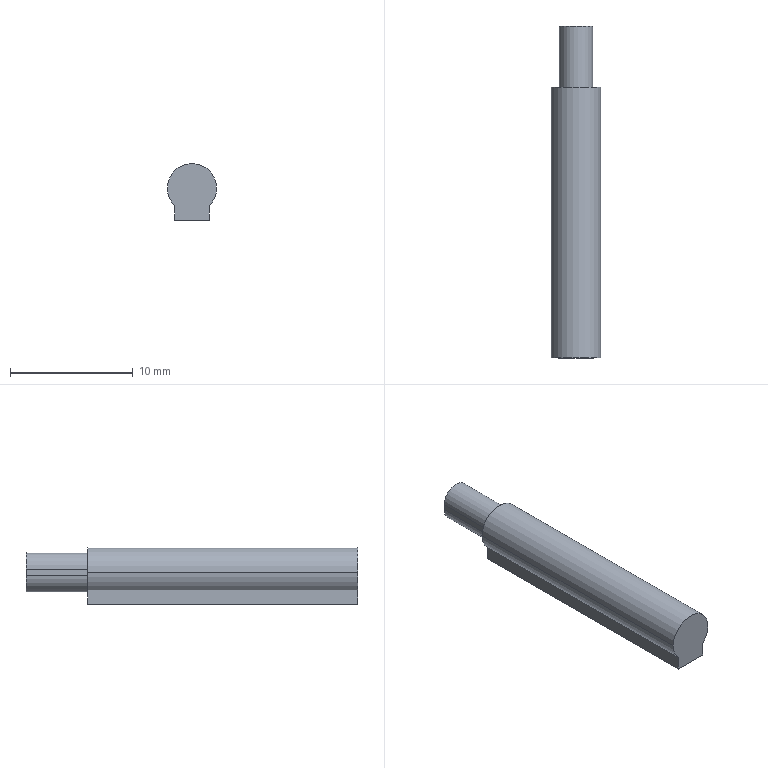Component | SolidWorks | RSDQA32-20DD-M9BL(0_0)-1_RSDQ_D-M9BL_SW(32)_2-1 | 1 solid | 16 faces | box 4 x 27 x 4.6 mm | volume 359 mm3 | plane 9 | cylinder 7 | commonest cylinder face diameters 4 x3 2.5 x2 2.7 x2
STEP:
#1=COLOUR_RGB('',0.7922,0.8196,0.9333);
#2=FILL_AREA_STYLE_COLOUR('',#1);
#3=FILL_AREA_STYLE('',(#2));
#4=SURFACE_STYLE_FILL_AREA(#3);
#5=SURFACE_SIDE_STYLE('',(#4));
#6=SURFACE_STYLE_USAGE(.BOTH.,#5);
#7=PRESENTATION_STYLE_ASSIGNMENT((#6));
#8=CARTESIAN_POINT('',(0.2128,-2.152,-1.666));
#9=VERTEX_POINT('',#8);
#10=CARTESIAN_POINT('',(0.1892,-2.152,-1.61));
#11=VERTEX_POINT('',#10);
#12=CARTESIAN_POINT('',(0.2679,-2.152,-1.61));
#13=DIRECTION('',(-0.,1.,0.));
#14=DIRECTION('',(1.,0.,0.));
#15=AXIS2_PLACEMENT_3D('',#12,#13,#14);
#16=CIRCLE('',#15,0.07874);
#17=EDGE_CURVE('',#9,#11,#16,.T.);
#18=ORIENTED_EDGE('',*,*,#17,.T.);
#19=CARTESIAN_POINT('',(0.1892,-1.286,-1.61));
#20=VERTEX_POINT('',#19);
#21=CARTESIAN_POINT('',(0.1892,-2.152,-1.61));
#22=DIRECTION('',(-0.,1.,0.));
#23=VECTOR('',#22,39.37);
#24=LINE('',#21,#23);
#25=EDGE_CURVE('',#11,#20,#24,.T.);
#26=ORIENTED_EDGE('',*,*,#25,.T.);
#27=CARTESIAN_POINT('',(0.2128,-1.286,-1.666));
#28=VERTEX_POINT('',#27);
#29=CARTESIAN_POINT('',(0.2679,-1.286,-1.61));
#30=DIRECTION('',(0.,-1.,-0.));
#31=DIRECTION('',(1.,0.,-0.));
#32=AXIS2_PLACEMENT_3D('',#29,#30,#31);
#33=CIRCLE('',#32,0.07874);
#34=EDGE_CURVE('',#20,#28,#33,.T.);
#35=ORIENTED_EDGE('',*,*,#34,.T.);
#36=CARTESIAN_POINT('',(0.2128,-2.152,-1.666));
#37=DIRECTION('',(0.,-1.,-0.));
#38=VECTOR('',#37,39.37);
#39=LINE('',#36,#38);
#40=EDGE_CURVE('',#28,#9,#39,.T.);
#41=ORIENTED_EDGE('',*,*,#40,.T.);
#42=EDGE_LOOP('',(#18,#26,#35,#41));
#43=FACE_OUTER_BOUND('',#42,.T.);
#44=CARTESIAN_POINT('',(0.2679,-2.152,-1.61));
#45=DIRECTION('',(-0.,1.,0.));
#46=DIRECTION('',(1.,0.,0.));
#47=AXIS2_PLACEMENT_3D('',#44,#45,#46);
#48=CYLINDRICAL_SURFACE('',#47,0.07874);
#49=ADVANCED_FACE('',(#43),#48,.T.);
#50=ORIENTED_EDGE('',*,*,#25,.F.);
#51=CARTESIAN_POINT('',(0.3466,-2.152,-1.61));
#52=VERTEX_POINT('',#51);
#53=CARTESIAN_POINT('',(0.2679,-2.152,-1.61));
#54=DIRECTION('',(-0.,1.,0.));
#55=DIRECTION('',(1.,0.,0.));
#56=AXIS2_PLACEMENT_3D('',#53,#54,#55);
#57=CIRCLE('',#56,0.07874);
#58=EDGE_CURVE('',#11,#52,#57,.T.);
#59=ORIENTED_EDGE('',*,*,#58,.T.);
#60=CARTESIAN_POINT('',(0.3466,-1.286,-1.61));
#61=VERTEX_POINT('',#60);
#62=CARTESIAN_POINT('',(0.3466,-2.152,-1.61));
#63=DIRECTION('',(-0.,1.,0.));
#64=VECTOR('',#63,39.37);
#65=LINE('',#62,#64);
#66=EDGE_CURVE('',#52,#61,#65,.T.);
#67=ORIENTED_EDGE('',*,*,#66,.T.);
#68=CARTESIAN_POINT('',(0.2679,-1.286,-1.61));
#69=DIRECTION('',(0.,-1.,-0.));
#70=DIRECTION('',(1.,0.,0.));
#71=AXIS2_PLACEMENT_3D('',#68,#69,#70);
#72=CIRCLE('',#71,0.07874);
#73=EDGE_CURVE('',#61,#20,#72,.T.);
#74=ORIENTED_EDGE('',*,*,#73,.T.);
#75=EDGE_LOOP('',(#50,#59,#67,#74));
#76=FACE_OUTER_BOUND('',#75,.T.);
#77=CARTESIAN_POINT('',(0.2679,-2.152,-1.61));
#78=DIRECTION('',(-0.,1.,0.));
#79=DIRECTION('',(1.,0.,0.));
#80=AXIS2_PLACEMENT_3D('',#77,#78,#79);
#81=CYLINDRICAL_SURFACE('',#80,0.07874);
#82=ADVANCED_FACE('',(#76),#81,.T.);
#83=CARTESIAN_POINT('',(0.3171,-2.073,-1.713));
#84=VERTEX_POINT('',#83);
#85=CARTESIAN_POINT('',(0.2187,-2.073,-1.713));
#86=VERTEX_POINT('',#85);
#87=CARTESIAN_POINT('',(0.2679,-2.073,-1.713));
#88=DIRECTION('',(0.,-0.,1.));
#89=DIRECTION('',(-1.,0.,0.));
#90=AXIS2_PLACEMENT_3D('',#87,#88,#89);
#91=CIRCLE('',#90,0.04921);
#92=EDGE_CURVE('',#84,#86,#91,.T.);
#93=ORIENTED_EDGE('',*,*,#92,.F.);
#94=CARTESIAN_POINT('',(0.3171,-2.073,-1.705));
#95=VERTEX_POINT('',#94);
#96=CARTESIAN_POINT('',(0.3171,-2.073,-1.713));
#97=DIRECTION('',(0.,-0.,1.));
#98=VECTOR('',#97,39.37);
#99=LINE('',#96,#98);
#100=EDGE_CURVE('',#84,#95,#99,.T.);
#101=ORIENTED_EDGE('',*,*,#100,.T.);
#102=CARTESIAN_POINT('',(0.2187,-2.073,-1.705));
#103=VERTEX_POINT('',#102);
#104=CARTESIAN_POINT('',(0.2679,-2.073,-1.705));
#105=DIRECTION('',(-0.,0.,-1.));
#106=DIRECTION('',(-1.,0.,0.));
#107=AXIS2_PLACEMENT_3D('',#104,#105,#106);
#108=CIRCLE('',#107,0.04921);
#109=EDGE_CURVE('',#103,#95,#108,.T.);
#110=ORIENTED_EDGE('',*,*,#109,.F.);
#111=CARTESIAN_POINT('',(0.2187,-2.073,-1.713));
#112=DIRECTION('',(0.,-0.,1.));
#113=VECTOR('',#112,39.37);
#114=LINE('',#111,#113);
#115=EDGE_CURVE('',#86,#103,#114,.T.);
#116=ORIENTED_EDGE('',*,*,#115,.F.);
#117=EDGE_LOOP('',(#93,#101,#110,#116));
#118=FACE_OUTER_BOUND('',#117,.T.);
#119=CARTESIAN_POINT('',(0.2679,-2.073,-1.713));
#120=DIRECTION('',(0.,-0.,1.));
#121=DIRECTION('',(-1.,0.,0.));
#122=AXIS2_PLACEMENT_3D('',#119,#120,#121);
#123=CYLINDRICAL_SURFACE('',#122,0.04921);
#124=ADVANCED_FACE('',(#118),#123,.F.);
#125=ORIENTED_EDGE('',*,*,#66,.F.);
#126=CARTESIAN_POINT('',(0.323,-2.152,-1.666));
#127=VERTEX_POINT('',#126);
#128=CARTESIAN_POINT('',(0.2679,-2.152,-1.61));
#129=DIRECTION('',(-0.,1.,0.));
#130=DIRECTION('',(1.,0.,0.));
#131=AXIS2_PLACEMENT_3D('',#128,#129,#130);
#132=CIRCLE('',#131,0.07874);
#133=EDGE_CURVE('',#52,#127,#132,.T.);
#134=ORIENTED_EDGE('',*,*,#133,.T.);
#135=CARTESIAN_POINT('',(0.323,-1.286,-1.666));
#136=VERTEX_POINT('',#135);
#137=CARTESIAN_POINT('',(0.323,-2.152,-1.666));
#138=DIRECTION('',(-0.,1.,0.));
#139=VECTOR('',#138,39.37);
#140=LINE('',#137,#139);
#141=EDGE_CURVE('',#127,#136,#140,.T.);
#142=ORIENTED_EDGE('',*,*,#141,.T.);
#143=CARTESIAN_POINT('',(0.2679,-1.286,-1.61));
#144=DIRECTION('',(0.,-1.,-0.));
#145=DIRECTION('',(1.,0.,-0.));
#146=AXIS2_PLACEMENT_3D('',#143,#144,#145);
#147=CIRCLE('',#146,0.07874);
#148=EDGE_CURVE('',#136,#61,#147,.T.);
#149=ORIENTED_EDGE('',*,*,#148,.T.);
#150=EDGE_LOOP('',(#125,#134,#142,#149));
#151=FACE_OUTER_BOUND('',#150,.T.);
#152=CARTESIAN_POINT('',(0.2679,-2.152,-1.61));
#153=DIRECTION('',(-0.,1.,0.));
#154=DIRECTION('',(1.,0.,0.));
#155=AXIS2_PLACEMENT_3D('',#152,#153,#154);
#156=CYLINDRICAL_SURFACE('',#155,0.07874);
#157=ADVANCED_FACE('',(#151),#156,.T.);
#158=CARTESIAN_POINT('',(0.323,-2.152,-1.713));
#159=VERTEX_POINT('',#158);
#160=CARTESIAN_POINT('',(0.323,-2.152,-1.713));
#161=DIRECTION('',(-0.,0.,-1.));
#162=VECTOR('',#161,39.37);
#163=LINE('',#160,#162);
#164=EDGE_CURVE('',#127,#159,#163,.T.);
#165=ORIENTED_EDGE('',*,*,#164,.T.);
#166=CARTESIAN_POINT('',(0.323,-1.286,-1.713));
#167=VERTEX_POINT('',#166);
#168=CARTESIAN_POINT('',(0.323,-2.152,-1.713));
#169=DIRECTION('',(-0.,1.,0.));
#170=VECTOR('',#169,39.37);
#171=LINE('',#168,#170);
#172=EDGE_CURVE('',#159,#167,#171,.T.);
#173=ORIENTED_EDGE('',*,*,#172,.T.);
#174=CARTESIAN_POINT('',(0.323,-1.286,-1.713));
#175=DIRECTION('',(0.,-0.,1.));
#176=VECTOR('',#175,39.37);
#177=LINE('',#174,#176);
#178=EDGE_CURVE('',#167,#136,#177,.T.);
#179=ORIENTED_EDGE('',*,*,#178,.T.);
#180=ORIENTED_EDGE('',*,*,#141,.F.);
#181=EDGE_LOOP('',(#165,#173,#179,#180));
#182=FACE_OUTER_BOUND('',#181,.T.);
#183=CARTESIAN_POINT('',(0.323,-2.152,-1.713));
#184=DIRECTION('',(1.,0.,-0.));
#185=DIRECTION('',(0.,-1.,-0.));
#186=AXIS2_PLACEMENT_3D('',#183,#184,#185);
#187=PLANE('',#186);
#188=ADVANCED_FACE('',(#182),#187,.T.);
#189=CARTESIAN_POINT('',(0.2128,-2.152,-1.713));
#190=VERTEX_POINT('',#189);
#191=CARTESIAN_POINT('',(0.2128,-2.152,-1.61));
#192=DIRECTION('',(0.,-0.,1.));
#193=VECTOR('',#192,39.37);
#194=LINE('',#191,#193);
#195=EDGE_CURVE('',#190,#9,#194,.T.);
#196=ORIENTED_EDGE('',*,*,#195,.F.);
#197=CARTESIAN_POINT('',(0.2679,-2.152,-1.713));
#198=DIRECTION('',(-1.,-0.,0.));
#199=VECTOR('',#198,39.37);
#200=LINE('',#197,#199);
#201=EDGE_CURVE('',#159,#190,#200,.T.);
#202=ORIENTED_EDGE('',*,*,#201,.F.);
#203=ORIENTED_EDGE('',*,*,#164,.F.);
#204=ORIENTED_EDGE('',*,*,#133,.F.);
#205=ORIENTED_EDGE('',*,*,#58,.F.);
#206=ORIENTED_EDGE('',*,*,#17,.F.);
#207=EDGE_LOOP('',(#196,#202,#203,#204,#205,#206));
#208=FACE_OUTER_BOUND('',#207,.T.);
#209=CARTESIAN_POINT('',(0.2679,-2.152,-1.61));
#210=DIRECTION('',(-0.,1.,0.));
#211=DIRECTION('',(1.,0.,-0.));
#212=AXIS2_PLACEMENT_3D('',#209,#210,#211);
#213=PLANE('',#212);
#214=ADVANCED_FACE('',(#208),#213,.F.);
#215=ORIENTED_EDGE('',*,*,#195,.T.);
#216=ORIENTED_EDGE('',*,*,#40,.F.);
#217=CARTESIAN_POINT('',(0.2128,-1.286,-1.713));
#218=VERTEX_POINT('',#217);
#219=CARTESIAN_POINT('',(0.2128,-1.286,-1.666));
#220=DIRECTION('',(-0.,0.,-1.));
#221=VECTOR('',#220,39.37);
#222=LINE('',#219,#221);
#223=EDGE_CURVE('',#28,#218,#222,.T.);
#224=ORIENTED_EDGE('',*,*,#223,.T.);
#225=CARTESIAN_POINT('',(0.2128,-2.152,-1.713));
#226=DIRECTION('',(0.,-1.,-0.));
#227=VECTOR('',#226,39.37);
#228=LINE('',#225,#227);
#229=EDGE_CURVE('',#218,#190,#228,.T.);
#230=ORIENTED_EDGE('',*,*,#229,.T.);
#231=EDGE_LOOP('',(#215,#216,#224,#230));
#232=FACE_OUTER_BOUND('',#231,.T.);
#233=CARTESIAN_POINT('',(0.2128,-2.152,-1.666));
#234=DIRECTION('',(-1.,-0.,0.));
#235=DIRECTION('',(-0.,1.,0.));
#236=AXIS2_PLACEMENT_3D('',#233,#234,#235);
#237=PLANE('',#236);
#238=ADVANCED_FACE('',(#232),#237,.T.);
#239=ORIENTED_EDGE('',*,*,#178,.F.);
#240=CARTESIAN_POINT('',(0.2679,-1.286,-1.713));
#241=DIRECTION('',(-1.,-0.,0.));
#242=VECTOR('',#241,39.37);
#243=LINE('',#240,#242);
#244=EDGE_CURVE('',#167,#218,#243,.T.);
#245=ORIENTED_EDGE('',*,*,#244,.T.);
#246=ORIENTED_EDGE('',*,*,#223,.F.);
#247=ORIENTED_EDGE('',*,*,#34,.F.);
#248=ORIENTED_EDGE('',*,*,#73,.F.);
#249=ORIENTED_EDGE('',*,*,#148,.F.);
#250=EDGE_LOOP('',(#239,#245,#246,#247,#248,#249));
#251=FACE_OUTER_BOUND('',#250,.T.);
#252=CARTESIAN_POINT('',(0.3211,-1.286,-1.6));
#253=VERTEX_POINT('',#252);
#254=CARTESIAN_POINT('',(0.3211,-1.286,-1.62));
#255=VERTEX_POINT('',#254);
#256=CARTESIAN_POINT('',(0.3211,-1.286,-1.62));
#257=DIRECTION('',(-0.,0.,-1.));
#258=VECTOR('',#257,39.37);
#259=LINE('',#256,#258);
#260=EDGE_CURVE('',#253,#255,#259,.T.);
#261=ORIENTED_EDGE('',*,*,#260,.F.);
#262=CARTESIAN_POINT('',(0.2148,-1.286,-1.6));
#263=VERTEX_POINT('',#262);
#264=CARTESIAN_POINT('',(0.2679,-1.286,-1.6));
#265=DIRECTION('',(0.,-1.,-0.));
#266=DIRECTION('',(1.,0.,0.));
#267=AXIS2_PLACEMENT_3D('',#264,#265,#266);
#268=CIRCLE('',#267,0.05315);
#269=EDGE_CURVE('',#253,#263,#268,.T.);
#270=ORIENTED_EDGE('',*,*,#269,.T.);
#271=CARTESIAN_POINT('',(0.2148,-1.286,-1.62));
#272=VERTEX_POINT('',#271);
#273=CARTESIAN_POINT('',(0.2148,-1.286,-1.6));
#274=DIRECTION('',(0.,-0.,1.));
#275=VECTOR('',#274,39.37);
#276=LINE('',#273,#275);
#277=EDGE_CURVE('',#272,#263,#276,.T.);
#278=ORIENTED_EDGE('',*,*,#277,.F.);
#279=CARTESIAN_POINT('',(0.2679,-1.286,-1.62));
#280=DIRECTION('',(0.,-1.,-0.));
#281=DIRECTION('',(1.,0.,0.));
#282=AXIS2_PLACEMENT_3D('',#279,#280,#281);
#283=CIRCLE('',#282,0.05315);
#284=EDGE_CURVE('',#272,#255,#283,.T.);
#285=ORIENTED_EDGE('',*,*,#284,.T.);
#286=EDGE_LOOP('',(#261,#270,#278,#285));
#287=FACE_BOUND('',#286,.T.);
#288=CARTESIAN_POINT('',(0.2679,-1.286,-1.61));
#289=DIRECTION('',(-0.,1.,0.));
#290=DIRECTION('',(1.,0.,-0.));
#291=AXIS2_PLACEMENT_3D('',#288,#289,#290);
#292=PLANE('',#291);
#293=ADVANCED_FACE('',(#251,#287),#292,.T.);
#294=ORIENTED_EDGE('',*,*,#201,.T.);
#295=ORIENTED_EDGE('',*,*,#229,.F.);
#296=ORIENTED_EDGE('',*,*,#244,.F.);
#297=ORIENTED_EDGE('',*,*,#172,.F.);
#298=EDGE_LOOP('',(#294,#295,#296,#297));
#299=FACE_OUTER_BOUND('',#298,.T.);
#300=CARTESIAN_POINT('',(0.2679,-2.073,-1.713));
#301=DIRECTION('',(0.,-0.,1.));
#302=DIRECTION('',(-1.,0.,0.));
#303=AXIS2_PLACEMENT_3D('',#300,#301,#302);
#304=CIRCLE('',#303,0.04921);
#305=EDGE_CURVE('',#86,#84,#304,.T.);
#306=ORIENTED_EDGE('',*,*,#305,.T.);
#307=ORIENTED_EDGE('',*,*,#92,.T.);
#308=EDGE_LOOP('',(#306,#307));
#309=FACE_BOUND('',#308,.T.);
#310=CARTESIAN_POINT('',(0.2128,-2.152,-1.713));
#311=DIRECTION('',(-0.,0.,-1.));
#312=DIRECTION('',(1.,0.,-0.));
#313=AXIS2_PLACEMENT_3D('',#310,#311,#312);
#314=PLANE('',#313);
#315=ADVANCED_FACE('',(#299,#309),#314,.T.);
#316=CARTESIAN_POINT('',(0.3211,-1.089,-1.6));
#317=VERTEX_POINT('',#316);
#318=CARTESIAN_POINT('',(0.2148,-1.089,-1.6));
#319=VERTEX_POINT('',#318);
#320=CARTESIAN_POINT('',(0.2679,-1.089,-1.6));
#321=DIRECTION('',(0.,-1.,-0.));
#322=DIRECTION('',(1.,0.,0.));
#323=AXIS2_PLACEMENT_3D('',#320,#321,#322);
#324=CIRCLE('',#323,0.05315);
#325=EDGE_CURVE('',#317,#319,#324,.T.);
#326=ORIENTED_EDGE('',*,*,#325,.T.);
#327=CARTESIAN_POINT('',(0.2148,-2.152,-1.6));
#328=DIRECTION('',(0.,-1.,-0.));
#329=VECTOR('',#328,39.37);
#330=LINE('',#327,#329);
#331=EDGE_CURVE('',#319,#263,#330,.T.);
#332=ORIENTED_EDGE('',*,*,#331,.T.);
#333=ORIENTED_EDGE('',*,*,#269,.F.);
#334=CARTESIAN_POINT('',(0.3211,-2.152,-1.6));
#335=DIRECTION('',(-0.,1.,0.));
#336=VECTOR('',#335,39.37);
#337=LINE('',#334,#336);
#338=EDGE_CURVE('',#253,#317,#337,.T.);
#339=ORIENTED_EDGE('',*,*,#338,.T.);
#340=EDGE_LOOP('',(#326,#332,#333,#339));
#341=FACE_OUTER_BOUND('',#340,.T.);
#342=CARTESIAN_POINT('',(0.2679,-2.152,-1.6));
#343=DIRECTION('',(-0.,1.,0.));
#344=DIRECTION('',(1.,0.,0.));
#345=AXIS2_PLACEMENT_3D('',#342,#343,#344);
#346=CYLINDRICAL_SURFACE('',#345,0.05315);
#347=ADVANCED_FACE('',(#341),#346,.T.);
#348=CARTESIAN_POINT('',(0.2148,-1.089,-1.62));
#349=VERTEX_POINT('',#348);
#350=CARTESIAN_POINT('',(0.3211,-1.089,-1.62));
#351=VERTEX_POINT('',#350);
#352=CARTESIAN_POINT('',(0.2679,-1.089,-1.62));
#353=DIRECTION('',(0.,-1.,-0.));
#354=DIRECTION('',(1.,0.,0.));
#355=AXIS2_PLACEMENT_3D('',#352,#353,#354);
#356=CIRCLE('',#355,0.05315);
#357=EDGE_CURVE('',#349,#351,#356,.T.);
#358=ORIENTED_EDGE('',*,*,#357,.T.);
#359=CARTESIAN_POINT('',(0.3211,-2.152,-1.62));
#360=DIRECTION('',(0.,-1.,-0.));
#361=VECTOR('',#360,39.37);
#362=LINE('',#359,#361);
#363=EDGE_CURVE('',#351,#255,#362,.T.);
#364=ORIENTED_EDGE('',*,*,#363,.T.);
#365=ORIENTED_EDGE('',*,*,#284,.F.);
#366=CARTESIAN_POINT('',(0.2148,-2.152,-1.62));
#367=DIRECTION('',(-0.,1.,0.));
#368=VECTOR('',#367,39.37);
#369=LINE('',#366,#368);
#370=EDGE_CURVE('',#272,#349,#369,.T.);
#371=ORIENTED_EDGE('',*,*,#370,.T.);
#372=EDGE_LOOP('',(#358,#364,#365,#371));
#373=FACE_OUTER_BOUND('',#372,.T.);
#374=CARTESIAN_POINT('',(0.2679,-2.152,-1.62));
#375=DIRECTION('',(-0.,1.,0.));
#376=DIRECTION('',(1.,0.,0.));
#377=AXIS2_PLACEMENT_3D('',#374,#375,#376);
#378=CYLINDRICAL_SURFACE('',#377,0.05315);
#379=ADVANCED_FACE('',(#373),#378,.T.);
#380=ORIENTED_EDGE('',*,*,#100,.F.);
#381=ORIENTED_EDGE('',*,*,#305,.F.);
#382=ORIENTED_EDGE('',*,*,#115,.T.);
#383=CARTESIAN_POINT('',(0.2679,-2.073,-1.705));
#384=DIRECTION('',(-0.,0.,-1.));
#385=DIRECTION('',(-1.,0.,0.));
#386=AXIS2_PLACEMENT_3D('',#383,#384,#385);
#387=CIRCLE('',#386,0.04921);
#388=EDGE_CURVE('',#95,#103,#387,.T.);
#389=ORIENTED_EDGE('',*,*,#388,.F.);
#390=EDGE_LOOP('',(#380,#381,#382,#389));
#391=FACE_OUTER_BOUND('',#390,.T.);
#392=CARTESIAN_POINT('',(0.2679,-2.073,-1.713));
#393=DIRECTION('',(0.,-0.,1.));
#394=DIRECTION('',(-1.,0.,0.));
#395=AXIS2_PLACEMENT_3D('',#392,#393,#394);
#396=CYLINDRICAL_SURFACE('',#395,0.04921);
#397=ADVANCED_FACE('',(#391),#396,.F.);
#398=CARTESIAN_POINT('',(0.2148,-1.089,-1.6));
#399=DIRECTION('',(-0.,0.,-1.));
#400=VECTOR('',#399,39.37);
#401=LINE('',#398,#400);
#402=EDGE_CURVE('',#319,#349,#401,.T.);
#403=ORIENTED_EDGE('',*,*,#402,.T.);
#404=ORIENTED_EDGE('',*,*,#370,.F.);
#405=ORIENTED_EDGE('',*,*,#277,.T.);
#406=ORIENTED_EDGE('',*,*,#331,.F.);
#407=EDGE_LOOP('',(#403,#404,#405,#406));
#408=FACE_OUTER_BOUND('',#407,.T.);
#409=CARTESIAN_POINT('',(0.2148,-2.152,-1.6));
#410=DIRECTION('',(-1.,-0.,0.));
#411=DIRECTION('',(-0.,1.,0.));
#412=AXIS2_PLACEMENT_3D('',#409,#410,#411);
#413=PLANE('',#412);
#414=ADVANCED_FACE('',(#408),#413,.T.);
#415=CARTESIAN_POINT('',(0.3211,-1.089,-1.61));
#416=DIRECTION('',(-0.,0.,-1.));
#417=VECTOR('',#416,39.37);
#418=LINE('',#415,#417);
#419=EDGE_CURVE('',#317,#351,#418,.T.);
#420=ORIENTED_EDGE('',*,*,#419,.T.);
#421=ORIENTED_EDGE('',*,*,#357,.F.);
#422=ORIENTED_EDGE('',*,*,#402,.F.);
#423=ORIENTED_EDGE('',*,*,#325,.F.);
#424=EDGE_LOOP('',(#420,#421,#422,#423));
#425=FACE_OUTER_BOUND('',#424,.T.);
#426=CARTESIAN_POINT('',(0.2679,-1.089,-1.61));
#427=DIRECTION('',(-0.,1.,0.));
#428=DIRECTION('',(1.,0.,-0.));
#429=AXIS2_PLACEMENT_3D('',#426,#427,#428);
#430=PLANE('',#429);
#431=ADVANCED_FACE('',(#425),#430,.T.);
#432=ORIENTED_EDGE('',*,*,#419,.F.);
#433=ORIENTED_EDGE('',*,*,#338,.F.);
#434=ORIENTED_EDGE('',*,*,#260,.T.);
#435=ORIENTED_EDGE('',*,*,#363,.F.);
#436=EDGE_LOOP('',(#432,#433,#434,#435));
#437=FACE_OUTER_BOUND('',#436,.T.);
#438=CARTESIAN_POINT('',(0.3211,-2.152,-1.62));
#439=DIRECTION('',(1.,0.,-0.));
#440=DIRECTION('',(0.,-1.,-0.));
#441=AXIS2_PLACEMENT_3D('',#438,#439,#440);
#442=PLANE('',#441);
#443=ADVANCED_FACE('',(#437),#442,.T.);
#444=ORIENTED_EDGE('',*,*,#109,.T.);
#445=ORIENTED_EDGE('',*,*,#388,.T.);
#446=EDGE_LOOP('',(#444,#445));
#447=FACE_OUTER_BOUND('',#446,.T.);
#448=CARTESIAN_POINT('',(0.2679,-2.152,-1.705));
#449=DIRECTION('',(-0.,0.,-1.));
#450=DIRECTION('',(1.,0.,-0.));
#451=AXIS2_PLACEMENT_3D('',#448,#449,#450);
#452=PLANE('',#451);
#453=ADVANCED_FACE('',(#447),#452,.T.);
#454=CLOSED_SHELL('',(#49,#82,#124,#157,#188,#214,#238,#293,#315,#347,#379,#397,#414,#431,#443,#453));
#455=MANIFOLD_SOLID_BREP('',#454);
#456=STYLED_ITEM('',(#7),#455);
#457=PRESENTATION_LAYER_ASSIGNMENT('','',(#456));
#458=CARTESIAN_POINT('',(0.,0.,0.));
#459=DIRECTION('',(0.,0.,1.));
#460=DIRECTION('',(1.,0.,0.));
#461=AXIS2_PLACEMENT_3D('',#458,#459,#460);
#462=(LENGTH_UNIT()NAMED_UNIT(*)SI_UNIT($,.METRE.));
#463=LENGTH_MEASURE_WITH_UNIT(LENGTH_MEASURE(0.0254),#462);
#464=DIMENSIONAL_EXPONENTS(1.,0.,0.,0.,0.,0.,0.);
#465=(CONVERSION_BASED_UNIT('',#463)LENGTH_UNIT()NAMED_UNIT(#464));
#466=UNCERTAINTY_MEASURE_WITH_UNIT(LENGTH_MEASURE(0.00001),#465,'','');
#467=(NAMED_UNIT(*)PLANE_ANGLE_UNIT()SI_UNIT($,.RADIAN.));
#468=(NAMED_UNIT(*)SI_UNIT($,.STERADIAN.)SOLID_ANGLE_UNIT());
#469=(GEOMETRIC_REPRESENTATION_CONTEXT(3)GLOBAL_UNCERTAINTY_ASSIGNED_CONTEXT((#466))GLOBAL_UNIT_ASSIGNED_CONTEXT((#465,#467,#468))REPRESENTATION_CONTEXT('',''));
#470=ADVANCED_BREP_SHAPE_REPRESENTATION('',(#455,#461),#469);
#471=(LENGTH_UNIT()NAMED_UNIT(*)SI_UNIT($,.METRE.));
#472=LENGTH_MEASURE_WITH_UNIT(LENGTH_MEASURE(0.0254),#471);
#473=DIMENSIONAL_EXPONENTS(1.,0.,0.,0.,0.,0.,0.);
#474=(CONVERSION_BASED_UNIT('',#472)LENGTH_UNIT()NAMED_UNIT(#473));
#475=UNCERTAINTY_MEASURE_WITH_UNIT(LENGTH_MEASURE(0.00001),#474,'','');
#476=(NAMED_UNIT(*)PLANE_ANGLE_UNIT()SI_UNIT($,.RADIAN.));
#477=(NAMED_UNIT(*)SI_UNIT($,.STERADIAN.)SOLID_ANGLE_UNIT());
#478=(GEOMETRIC_REPRESENTATION_CONTEXT(3)GLOBAL_UNCERTAINTY_ASSIGNED_CONTEXT((#475))GLOBAL_UNIT_ASSIGNED_CONTEXT((#474,#476,#477))REPRESENTATION_CONTEXT('',''));
#479=MECHANICAL_DESIGN_GEOMETRIC_PRESENTATION_REPRESENTATION('',(#456),#478);